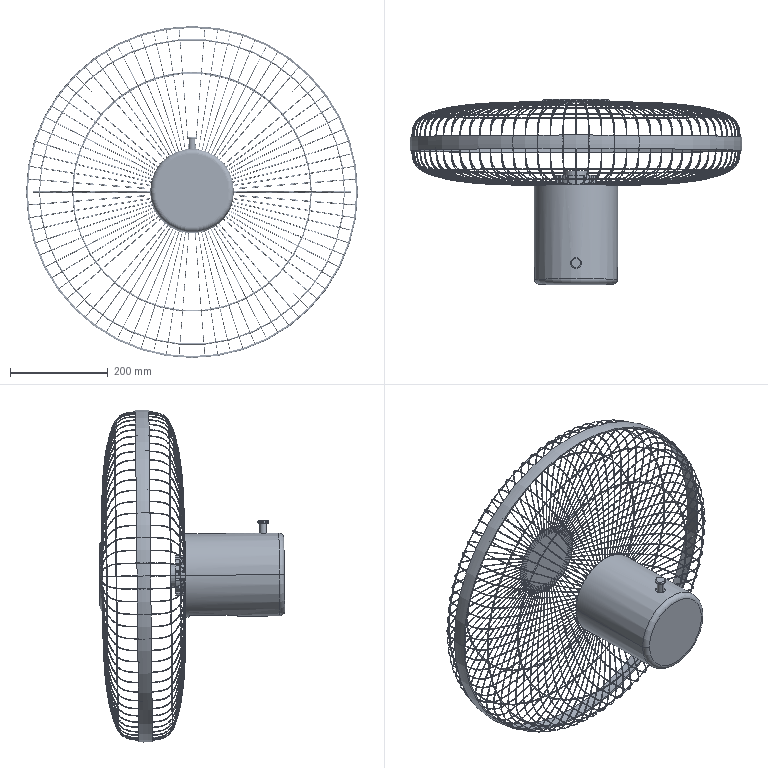Component | NX | OUTER_COVER | 5 solids | 863 faces | volume 1342051 mm3 | spline 326 | plane 288 | torus 195 | cylinder 48 | cone 6 | commonest cylinder face diameters 1 x18 75 x15 22 x2 13.5 x2 20 x2 45 x2 8 x2 160 x2